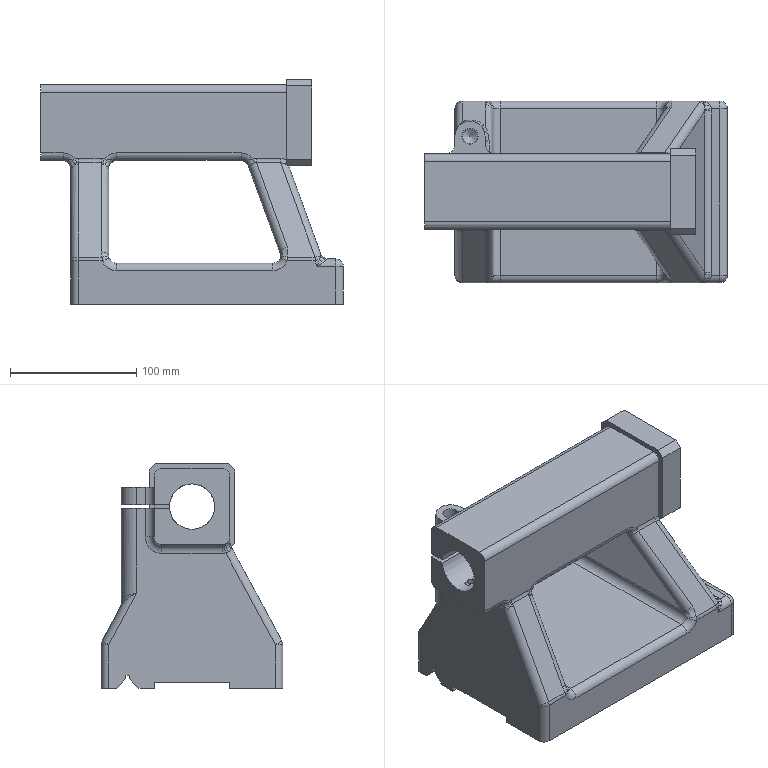Component | NX | FRAME | 1 solid | 178 faces | volume 2053409 mm3 | plane 58 | cylinder 53 | spline 38 | torus 13 | sphere 11 | cone 5 | commonest cylinder face diameters 12 x34 14 x10 7.76 x4 24 x2 36 x1 13 x1 6 x1